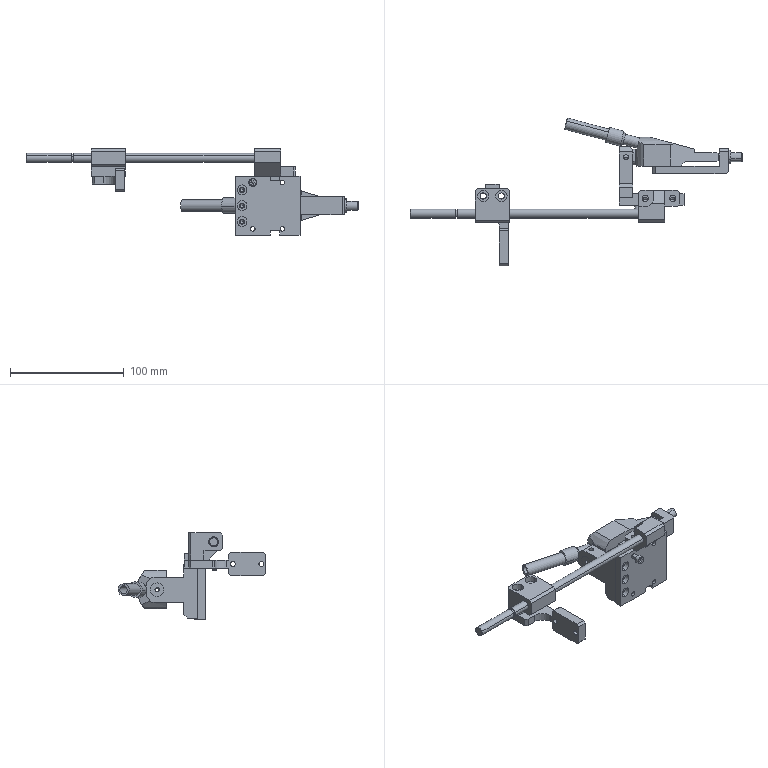Assembly | SolidWorks | mm | 13 component files | 13 solids | 351 faces | box 292 x 130.1 x 76.04 mm | volume 130272 mm3 | plane 172 | cylinder 143 | cone 36 | commonest cylinder face diameters 5.5 x14 4.2 x14 3.3 x14 8 x12 10 x10 4.5 x10 4 x10 12 x9
Bill of materials:
004CylinderConnectionBlock | 1 |  | Stepped prismatic block, roughly L-shaped: a wider head carrying two parallel through-holes and a small rectangular tab, joined by a concave radiused transition to a narrower arm that carries two through-holes running crosswise; corners are chamfered.
005SliderAdapter | 1 |  | Thick rectangular plate with rectangular notches centered on two opposite edges, a row of three larger through-holes along one edge, four smaller through-holes near the corners, and two holes drilled into one edge face.
006GuideSeat | 1 |  | Compact rectangular block with two parallel vertical through-holes from the top face, one larger cross hole through a side face, a chamfered edge, and a stepped rectangular projection or rabbet along the bottom.
007GuideRod | 1 |  | Long slender cylindrical rod or tube with a small circumferential groove near one end. The end view shows a central bore or recess with a conical bottom.
009BearingHousing | 1 |  | T-shaped bracket block: a vertical bar with three holes in its side face, and a horizontal arm with a chamfered end that has a large through-bore plus a small hole in its top face.
015GuideRodHolder | 1 |  | Stepped, offset block: a main rectangular body with a chamfered edge and a horizontal through-hole, plus a lower, narrower lug with a vertical through-hole. One view shows an angled (beveled) profile.
016WindShieldHolder | 1 |  | L-shaped bar with chamfered corners: a long arm with two transverse through-holes, and a short perpendicular leg with one large through-bore and a smaller hole that meets the bore.
017NailOutlet | 1 |  | Hollow, axially symmetric stepped sleeve: a larger-diameter section, a thin raised collar or flange, and a smaller-diameter section with a chamfered end. A through-bore runs along the axis, with a counterbore or chamfer at one end.
Connector | 1 |  | Hollow, axially symmetric stepped body: a large end section, a circumferential neck or groove, a second shoulder, a hex-like or flatted collar, a long smaller-diameter shank, and a short, even smaller tip. A central bore runs through.
M3Jaw | 1 |  | Tapered, wedge-like housing or nose block: a wider rounded body narrowing through angled faces to a smaller rectangular tip, with two holes on the broad face, a small hole at the tip, and a stepped internal cavity seen from the wide end.
AirTube | 1 |  | Plain straight cylindrical tube with a uniform outside diameter and a concentric through-bore.
ScrewFeedConnector | 1 |  | Hollow stepped cylindrical reducer-like shape: a larger-diameter section joined by a conical transition to a longer smaller-diameter section, with a concentric through-bore.
SocketHeadCapScrew_M4_16[GB_T70.1-2000] | 1 | Cobalt | Headed cylindrical pin shaped like a socket-head cap screw: a short cylindrical head with a hexagonal socket recess in its top face, and a long smooth cylindrical shank with a chamfered end. Threads are not modeled.
Mates:
1. concentric | 015GuideRodHolder-1 face at (30.76, 24.924, 53.04) dir (1, 0, 0) r 2.75 | 007GuideRod-2 face at (26.76, 24.924, 53.04) dir (1, 0, 0) r 2.1
2. coincident | 015GuideRodHolder-1 face at (26.76, 24.924, 53.04) dir (-1, 0, 0) | 007GuideRod-2 face at (26.76, 24.924, 53.04) dir (1, 0, 0)
3. distance | Connector-1 face at (4.76, 74.679, 11) dir (1, 0, 0) | M3Jaw-1 face at (5.76, 92.179, -6) dir (-1, 0, 0)
4. concentric | M3Jaw-1 face at (5.76, 74.679, 11) dir (-1, 0, 0) r 3.9 | Connector-1 face at (4.76, 74.679, 11) dir (1, 0, 0) r 3.9
5. concentric | M3Jaw-1 face at (27.76, 66.679, 11) dir (0, -1, 0) r 1.65 | 016WindShieldHolder-1 face at (27.76, 60.179, 11) dir (0, -1, 0) r 2.25
6. concentric | M3Jaw-1 face at (39.76, 66.679, 11) dir (0, -1, 0) r 1.65 | 016WindShieldHolder-1 face at (39.76, 60.179, 11) dir (0, -1, 0) r 2.25
7. coincident | M3Jaw-1 face at (41.76, 66.679, 11) dir (0, -1, 0) | 016WindShieldHolder-1 face at (19.76, 66.679, 19) dir (0, 1, 0)
8. concentric | 016WindShieldHolder-1 face at (19.76, 74.679, 11) dir (1, 0, 0) r 5 | 017NailOutlet-1 face at (86.76, 74.679, 11) dir (-1, 0, 0) r 5
9. coincident | 016WindShieldHolder-1 face at (86.76, 60.179, 3) dir (1, 0, 0) | 017NailOutlet-1 face at (86.76, 74.679, 11) dir (-1, 0, 0)
10. concentric | M3Jaw-1 face at (16.411, 84.726, 11) dir (-0.9659, 0.2588, 0) r 4.5 | ScrewFeedConnectorAssembly-1/ScrewFeedConnector-1 face at (17.909, 84.325, 11) dir (0.9659, -0.2588, 0) r 4.5
11. coincident | M3Jaw-1 face at (16.411, 84.726, 11) dir (-0.9659, 0.2588, 0) | ScrewFeedConnectorAssembly-1/ScrewFeedConnector-1 face at (16.339, 84.455, 14.037) dir (0.9659, -0.2588, 0)
12. concentric | 009BearingHousing-1 face at (-9.24, 74.679, 11) dir (1, 0, 0) r 6 | Connector-1 face at (2.76, 74.679, 11) dir (-1, 0, 0) r 6
13. coincident | 009BearingHousing-1 face at (-9.24, 61.679, 11) dir (-1, 0, 0) | Connector-1 face at (-9.24, 74.679, 11) dir (-1, 0, 0)
14. concentric | 005SliderAdapter-1 face at (-3.24, 32.179, 11) dir (0, -1, 0) r 2.25 | 009BearingHousing-1 face at (-3.24, 39.179, 11) dir (0, -1, 0) r 1.65
15. coincident | 005SliderAdapter-1 face at (2.76, 42.179, 37) dir (-1, 0, 0) | 009BearingHousing-1 face at (2.76, 61.679, 11) dir (1, 0, 0)
16. coincident | 005SliderAdapter-1 face at (-9.24, 39.179, 37) dir (0, 1, 0) | 009BearingHousing-1 face at (2.76, 39.179, 36) dir (0, -1, 0)
17. concentric | 005SliderAdapter-1 face at (6.26, 32.179, 31.5) dir (0, -1, 0) r 2 | SocketHeadCapScrew_M4_16[GB_T70.1-2000]-1 face at (6.26, 42.179, 31.5) dir (0, -1, 0) r 2
18. coincident | 015GuideRodHolder-1 face at (21.76, 45.424, 33.04) dir (-1, 0, 0) | 005SliderAdapter-1 face at (21.76, 32.179, 37) dir (1, 0, 0)
19. concentric | 006GuideSeat-3 face at (-135.796, 24.924, 53.04) dir (1, 0, 0) r 4.5 | 007GuideRod-2 face at (26.76, 24.924, 53.04) dir (-1, 0, 0) r 4
20. coincident | 004CylinderConnectionBlock-3 face at (-106.796, 46.924, 37.04) dir (0, 0, 1) | 006GuideSeat-3 face at (-135.796, 16.924, 37.04) dir (0, 0, -1)
21. concentric | 004CylinderConnectionBlock-3 face at (-128.796, 40.424, 44.04) dir (0, 0, -1) r 2.65 | 006GuideSeat-3 face at (-128.796, 40.424, 61.04) dir (0, 0, 1) r 2.75
22. concentric | 004CylinderConnectionBlock-3 face at (-112.796, 40.424, 44.04) dir (0, 0, -1) r 2.65 | 006GuideSeat-3 face at (-112.796, 40.424, 61.04) dir (0, 0, 1) r 2.75
23. coincident | ScrewFeedConnector-1 face at (0.5782, 3.545, 0) dir (0, 1, 0) | AirTube-3 face at (-6.172, 3.545, 0) dir (0, -1, 0)